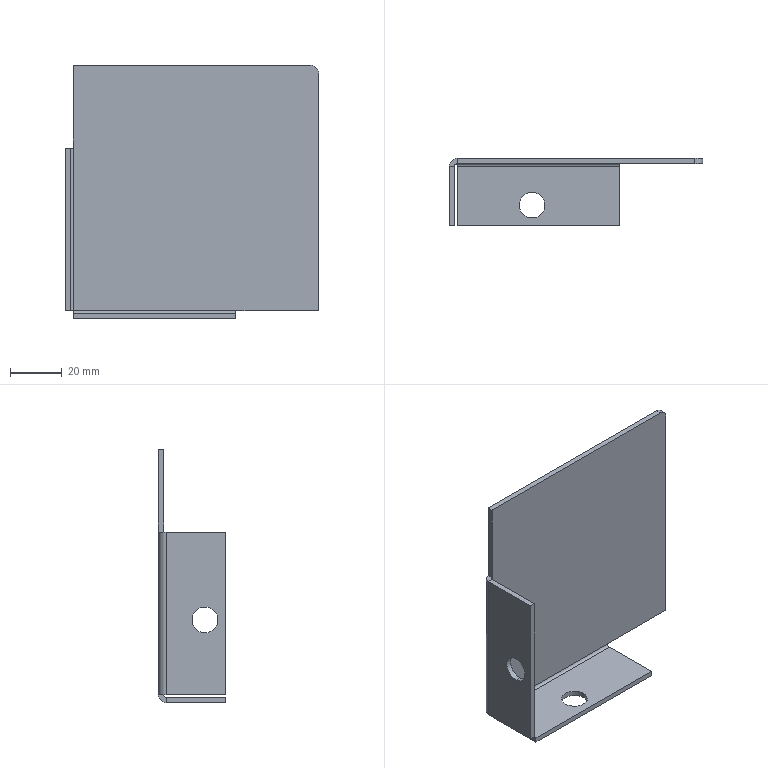Component | SolidWorks | ColumnBlockingPlate-2 | 1 solid | 29 faces | box 98 x 26 x 98 mm | volume 24320 mm3 | plane 20 | cylinder 9 | commonest cylinder face diameters 10 x4 6 x3 2 x2
STEP:
#1=CARTESIAN_POINT('',(85.767,85.53,45.831));
#2=VERTEX_POINT('',#1);
#3=CARTESIAN_POINT('',(85.767,85.53,46.225));
#4=VERTEX_POINT('',#3);
#5=CARTESIAN_POINT('',(85.767,85.53,46.028));
#6=DIRECTION('',(-1.,0.,0.));
#7=DIRECTION('',(0.,-1.,0.));
#8=AXIS2_PLACEMENT_3D('',#5,#6,#7);
#9=CIRCLE('',#8,0.1969);
#10=EDGE_CURVE('',#2,#4,#9,.T.);
#11=ORIENTED_EDGE('',*,*,#10,.F.);
#12=CARTESIAN_POINT('',(85.688,85.53,45.831));
#13=VERTEX_POINT('',#12);
#14=CARTESIAN_POINT('',(85.688,85.53,45.831));
#15=DIRECTION('',(-1.,0.,0.));
#16=VECTOR('',#15,39.37);
#17=LINE('',#14,#16);
#18=EDGE_CURVE('',#2,#13,#17,.T.);
#19=ORIENTED_EDGE('',*,*,#18,.T.);
#20=CARTESIAN_POINT('',(85.688,85.53,46.225));
#21=VERTEX_POINT('',#20);
#22=CARTESIAN_POINT('',(85.688,85.53,46.028));
#23=DIRECTION('',(-1.,0.,0.));
#24=DIRECTION('',(0.,0.,1.));
#25=AXIS2_PLACEMENT_3D('',#22,#23,#24);
#26=CIRCLE('',#25,0.1969);
#27=EDGE_CURVE('',#13,#21,#26,.T.);
#28=ORIENTED_EDGE('',*,*,#27,.T.);
#29=CARTESIAN_POINT('',(85.688,85.53,46.225));
#30=DIRECTION('',(-1.,0.,0.));
#31=VECTOR('',#30,39.37);
#32=LINE('',#29,#31);
#33=EDGE_CURVE('',#4,#21,#32,.T.);
#34=ORIENTED_EDGE('',*,*,#33,.F.);
#35=EDGE_LOOP('',(#11,#19,#28,#34));
#36=FACE_OUTER_BOUND('',#35,.T.);
#37=CARTESIAN_POINT('',(85.688,85.53,46.028));
#38=DIRECTION('',(-1.,0.,0.));
#39=DIRECTION('',(0.,0.,1.));
#40=AXIS2_PLACEMENT_3D('',#37,#38,#39);
#41=CYLINDRICAL_SURFACE('',#40,0.1969);
#42=ADVANCED_FACE('',(#36),#41,.F.);
#43=CARTESIAN_POINT('',(87.145,85.53,44.847));
#44=VERTEX_POINT('',#43);
#45=CARTESIAN_POINT('',(86.751,85.53,44.847));
#46=VERTEX_POINT('',#45);
#47=CARTESIAN_POINT('',(86.948,85.53,44.847));
#48=DIRECTION('',(-0.,0.,-1.));
#49=DIRECTION('',(0.,-1.,0.));
#50=AXIS2_PLACEMENT_3D('',#47,#48,#49);
#51=CIRCLE('',#50,0.1969);
#52=EDGE_CURVE('',#44,#46,#51,.T.);
#53=ORIENTED_EDGE('',*,*,#52,.F.);
#54=CARTESIAN_POINT('',(87.145,85.53,44.768));
#55=VERTEX_POINT('',#54);
#56=CARTESIAN_POINT('',(87.145,85.53,44.768));
#57=DIRECTION('',(-0.,0.,-1.));
#58=VECTOR('',#57,39.37);
#59=LINE('',#56,#58);
#60=EDGE_CURVE('',#44,#55,#59,.T.);
#61=ORIENTED_EDGE('',*,*,#60,.T.);
#62=CARTESIAN_POINT('',(86.751,85.53,44.768));
#63=VERTEX_POINT('',#62);
#64=CARTESIAN_POINT('',(86.948,85.53,44.768));
#65=DIRECTION('',(-0.,0.,-1.));
#66=DIRECTION('',(-1.,0.,0.));
#67=AXIS2_PLACEMENT_3D('',#64,#65,#66);
#68=CIRCLE('',#67,0.1969);
#69=EDGE_CURVE('',#55,#63,#68,.T.);
#70=ORIENTED_EDGE('',*,*,#69,.T.);
#71=CARTESIAN_POINT('',(86.751,85.53,44.768));
#72=DIRECTION('',(-0.,0.,-1.));
#73=VECTOR('',#72,39.37);
#74=LINE('',#71,#73);
#75=EDGE_CURVE('',#46,#63,#74,.T.);
#76=ORIENTED_EDGE('',*,*,#75,.F.);
#77=EDGE_LOOP('',(#53,#61,#70,#76));
#78=FACE_OUTER_BOUND('',#77,.T.);
#79=CARTESIAN_POINT('',(86.948,85.53,44.768));
#80=DIRECTION('',(-0.,0.,-1.));
#81=DIRECTION('',(-1.,0.,0.));
#82=AXIS2_PLACEMENT_3D('',#79,#80,#81);
#83=CYLINDRICAL_SURFACE('',#82,0.1969);
#84=ADVANCED_FACE('',(#78),#83,.F.);
#85=CARTESIAN_POINT('',(85.806,86.239,44.886));
#86=VERTEX_POINT('',#85);
#87=CARTESIAN_POINT('',(85.806,86.239,47.366));
#88=VERTEX_POINT('',#87);
#89=CARTESIAN_POINT('',(85.806,86.239,44.768));
#90=DIRECTION('',(0.,0.,1.));
#91=VECTOR('',#90,39.37);
#92=LINE('',#89,#91);
#93=EDGE_CURVE('',#86,#88,#92,.T.);
#94=ORIENTED_EDGE('',*,*,#93,.F.);
#95=CARTESIAN_POINT('',(85.688,86.12,44.886));
#96=VERTEX_POINT('',#95);
#97=CARTESIAN_POINT('',(85.806,86.12,44.886));
#98=DIRECTION('',(0.,0.,1.));
#99=DIRECTION('',(-1.,0.,0.));
#100=AXIS2_PLACEMENT_3D('',#97,#98,#99);
#101=CIRCLE('',#100,0.1181);
#102=EDGE_CURVE('',#86,#96,#101,.T.);
#103=ORIENTED_EDGE('',*,*,#102,.T.);
#104=CARTESIAN_POINT('',(85.688,86.12,47.366));
#105=VERTEX_POINT('',#104);
#106=CARTESIAN_POINT('',(85.688,86.12,44.768));
#107=DIRECTION('',(-0.,0.,-1.));
#108=VECTOR('',#107,39.37);
#109=LINE('',#106,#108);
#110=EDGE_CURVE('',#105,#96,#109,.T.);
#111=ORIENTED_EDGE('',*,*,#110,.F.);
#112=CARTESIAN_POINT('',(85.806,86.12,47.366));
#113=DIRECTION('',(0.,0.,1.));
#114=DIRECTION('',(1.,0.,0.));
#115=AXIS2_PLACEMENT_3D('',#112,#113,#114);
#116=CIRCLE('',#115,0.1181);
#117=EDGE_CURVE('',#88,#105,#116,.T.);
#118=ORIENTED_EDGE('',*,*,#117,.F.);
#119=EDGE_LOOP('',(#94,#103,#111,#118));
#120=FACE_OUTER_BOUND('',#119,.T.);
#121=CARTESIAN_POINT('',(85.806,86.12,44.768));
#122=DIRECTION('',(-0.,0.,-1.));
#123=DIRECTION('',(-1.,0.,0.));
#124=AXIS2_PLACEMENT_3D('',#121,#122,#123);
#125=CYLINDRICAL_SURFACE('',#124,0.1181);
#126=ADVANCED_FACE('',(#120),#125,.T.);
#127=CARTESIAN_POINT('',(85.806,86.16,44.886));
#128=VERTEX_POINT('',#127);
#129=CARTESIAN_POINT('',(85.767,86.12,44.886));
#130=VERTEX_POINT('',#129);
#131=CARTESIAN_POINT('',(85.806,86.12,44.886));
#132=DIRECTION('',(0.,-0.,1.));
#133=DIRECTION('',(0.,1.,0.));
#134=AXIS2_PLACEMENT_3D('',#131,#132,#133);
#135=CIRCLE('',#134,0.03937);
#136=EDGE_CURVE('',#128,#130,#135,.T.);
#137=ORIENTED_EDGE('',*,*,#136,.F.);
#138=CARTESIAN_POINT('',(85.806,86.16,47.366));
#139=VERTEX_POINT('',#138);
#140=CARTESIAN_POINT('',(85.806,86.16,44.768));
#141=DIRECTION('',(0.,0.,1.));
#142=VECTOR('',#141,39.37);
#143=LINE('',#140,#142);
#144=EDGE_CURVE('',#128,#139,#143,.T.);
#145=ORIENTED_EDGE('',*,*,#144,.T.);
#146=CARTESIAN_POINT('',(85.767,86.12,47.366));
#147=VERTEX_POINT('',#146);
#148=CARTESIAN_POINT('',(85.806,86.12,47.366));
#149=DIRECTION('',(-0.,0.,-1.));
#150=DIRECTION('',(1.,0.,0.));
#151=AXIS2_PLACEMENT_3D('',#148,#149,#150);
#152=CIRCLE('',#151,0.03937);
#153=EDGE_CURVE('',#147,#139,#152,.T.);
#154=ORIENTED_EDGE('',*,*,#153,.F.);
#155=CARTESIAN_POINT('',(85.767,86.12,48.626));
#156=DIRECTION('',(-0.,0.,-1.));
#157=VECTOR('',#156,39.37);
#158=LINE('',#155,#157);
#159=EDGE_CURVE('',#147,#130,#158,.T.);
#160=ORIENTED_EDGE('',*,*,#159,.T.);
#161=EDGE_LOOP('',(#137,#145,#154,#160));
#162=FACE_OUTER_BOUND('',#161,.T.);
#163=CARTESIAN_POINT('',(85.806,86.12,44.768));
#164=DIRECTION('',(-0.,0.,-1.));
#165=DIRECTION('',(-1.,0.,0.));
#166=AXIS2_PLACEMENT_3D('',#163,#164,#165);
#167=CYLINDRICAL_SURFACE('',#166,0.03937);
#168=ADVANCED_FACE('',(#162),#167,.F.);
#169=CARTESIAN_POINT('',(85.688,85.53,46.028));
#170=DIRECTION('',(-1.,0.,0.));
#171=DIRECTION('',(0.,0.,1.));
#172=AXIS2_PLACEMENT_3D('',#169,#170,#171);
#173=CIRCLE('',#172,0.1969);
#174=EDGE_CURVE('',#21,#13,#173,.T.);
#175=ORIENTED_EDGE('',*,*,#174,.F.);
#176=ORIENTED_EDGE('',*,*,#27,.F.);
#177=EDGE_LOOP('',(#175,#176));
#178=FACE_BOUND('',#177,.T.);
#179=ORIENTED_EDGE('',*,*,#110,.T.);
#180=CARTESIAN_POINT('',(85.688,85.215,44.886));
#181=VERTEX_POINT('',#180);
#182=CARTESIAN_POINT('',(85.688,86.16,44.886));
#183=DIRECTION('',(-0.,-1.,0.));
#184=VECTOR('',#183,39.37);
#185=LINE('',#182,#184);
#186=EDGE_CURVE('',#96,#181,#185,.T.);
#187=ORIENTED_EDGE('',*,*,#186,.T.);
#188=CARTESIAN_POINT('',(85.688,85.215,47.366));
#189=VERTEX_POINT('',#188);
#190=CARTESIAN_POINT('',(85.688,85.215,44.768));
#191=DIRECTION('',(-0.,0.,-1.));
#192=VECTOR('',#191,39.37);
#193=LINE('',#190,#192);
#194=EDGE_CURVE('',#189,#181,#193,.T.);
#195=ORIENTED_EDGE('',*,*,#194,.F.);
#196=CARTESIAN_POINT('',(85.688,86.12,47.366));
#197=DIRECTION('',(-0.,-1.,0.));
#198=VECTOR('',#197,39.37);
#199=LINE('',#196,#198);
#200=EDGE_CURVE('',#105,#189,#199,.T.);
#201=ORIENTED_EDGE('',*,*,#200,.F.);
#202=EDGE_LOOP('',(#179,#187,#195,#201));
#203=FACE_OUTER_BOUND('',#202,.T.);
#204=CARTESIAN_POINT('',(85.688,86.16,44.768));
#205=DIRECTION('',(-1.,0.,0.));
#206=DIRECTION('',(-0.,-1.,0.));
#207=AXIS2_PLACEMENT_3D('',#204,#205,#206);
#208=PLANE('',#207);
#209=ADVANCED_FACE('',(#178,#203),#208,.T.);
#210=CARTESIAN_POINT('',(85.767,85.53,46.028));
#211=DIRECTION('',(-1.,0.,0.));
#212=DIRECTION('',(0.,-1.,0.));
#213=AXIS2_PLACEMENT_3D('',#210,#211,#212);
#214=CIRCLE('',#213,0.1969);
#215=EDGE_CURVE('',#4,#2,#214,.T.);
#216=ORIENTED_EDGE('',*,*,#215,.T.);
#217=ORIENTED_EDGE('',*,*,#10,.T.);
#218=EDGE_LOOP('',(#216,#217));
#219=FACE_BOUND('',#218,.T.);
#220=CARTESIAN_POINT('',(85.767,85.215,44.886));
#221=VERTEX_POINT('',#220);
#222=CARTESIAN_POINT('',(85.767,86.12,44.886));
#223=DIRECTION('',(-0.,-1.,-0.));
#224=VECTOR('',#223,39.37);
#225=LINE('',#222,#224);
#226=EDGE_CURVE('',#130,#221,#225,.T.);
#227=ORIENTED_EDGE('',*,*,#226,.F.);
#228=ORIENTED_EDGE('',*,*,#159,.F.);
#229=CARTESIAN_POINT('',(85.767,85.215,47.366));
#230=VERTEX_POINT('',#229);
#231=CARTESIAN_POINT('',(85.767,85.215,47.366));
#232=DIRECTION('',(0.,1.,-0.));
#233=VECTOR('',#232,39.37);
#234=LINE('',#231,#233);
#235=EDGE_CURVE('',#230,#147,#234,.T.);
#236=ORIENTED_EDGE('',*,*,#235,.F.);
#237=CARTESIAN_POINT('',(85.767,85.215,44.768));
#238=DIRECTION('',(-0.,0.,-1.));
#239=VECTOR('',#238,39.37);
#240=LINE('',#237,#239);
#241=EDGE_CURVE('',#230,#221,#240,.T.);
#242=ORIENTED_EDGE('',*,*,#241,.T.);
#243=EDGE_LOOP('',(#227,#228,#236,#242));
#244=FACE_OUTER_BOUND('',#243,.T.);
#245=CARTESIAN_POINT('',(85.767,86.16,44.768));
#246=DIRECTION('',(-1.,0.,0.));
#247=DIRECTION('',(-0.,-1.,0.));
#248=AXIS2_PLACEMENT_3D('',#245,#246,#247);
#249=PLANE('',#248);
#250=ADVANCED_FACE('',(#219,#244),#249,.F.);
#251=ORIENTED_EDGE('',*,*,#194,.T.);
#252=CARTESIAN_POINT('',(85.767,85.215,44.886));
#253=DIRECTION('',(-1.,0.,0.));
#254=VECTOR('',#253,39.37);
#255=LINE('',#252,#254);
#256=EDGE_CURVE('',#221,#181,#255,.T.);
#257=ORIENTED_EDGE('',*,*,#256,.F.);
#258=ORIENTED_EDGE('',*,*,#241,.F.);
#259=CARTESIAN_POINT('',(85.688,85.215,47.366));
#260=DIRECTION('',(1.,-0.,-0.));
#261=VECTOR('',#260,39.37);
#262=LINE('',#259,#261);
#263=EDGE_CURVE('',#189,#230,#262,.T.);
#264=ORIENTED_EDGE('',*,*,#263,.F.);
#265=EDGE_LOOP('',(#251,#257,#258,#264));
#266=FACE_OUTER_BOUND('',#265,.T.);
#267=CARTESIAN_POINT('',(85.688,85.215,44.768));
#268=DIRECTION('',(-0.,-1.,0.));
#269=DIRECTION('',(1.,-0.,-0.));
#270=AXIS2_PLACEMENT_3D('',#267,#268,#269);
#271=PLANE('',#270);
#272=ADVANCED_FACE('',(#266),#271,.T.);
#273=ORIENTED_EDGE('',*,*,#235,.T.);
#274=CARTESIAN_POINT('',(85.767,86.12,47.366));
#275=DIRECTION('',(-1.,0.,0.));
#276=VECTOR('',#275,39.37);
#277=LINE('',#274,#276);
#278=EDGE_CURVE('',#147,#105,#277,.T.);
#279=ORIENTED_EDGE('',*,*,#278,.T.);
#280=ORIENTED_EDGE('',*,*,#200,.T.);
#281=ORIENTED_EDGE('',*,*,#263,.T.);
#282=EDGE_LOOP('',(#273,#279,#280,#281));
#283=FACE_OUTER_BOUND('',#282,.T.);
#284=CARTESIAN_POINT('',(85.806,86.12,47.366));
#285=DIRECTION('',(0.,0.,1.));
#286=DIRECTION('',(1.,0.,-0.));
#287=AXIS2_PLACEMENT_3D('',#284,#285,#286);
#288=PLANE('',#287);
#289=ADVANCED_FACE('',(#283),#288,.T.);
#290=CARTESIAN_POINT('',(88.286,85.215,44.768));
#291=VERTEX_POINT('',#290);
#292=CARTESIAN_POINT('',(88.286,86.12,44.768));
#293=VERTEX_POINT('',#292);
#294=CARTESIAN_POINT('',(88.286,85.215,44.768));
#295=DIRECTION('',(0.,1.,0.));
#296=VECTOR('',#295,39.37);
#297=LINE('',#294,#296);
#298=EDGE_CURVE('',#291,#293,#297,.T.);
#299=ORIENTED_EDGE('',*,*,#298,.T.);
#300=CARTESIAN_POINT('',(88.286,86.12,44.847));
#301=VERTEX_POINT('',#300);
#302=CARTESIAN_POINT('',(88.286,86.12,44.768));
#303=DIRECTION('',(0.,-0.,1.));
#304=VECTOR('',#303,39.37);
#305=LINE('',#302,#304);
#306=EDGE_CURVE('',#293,#301,#305,.T.);
#307=ORIENTED_EDGE('',*,*,#306,.T.);
#308=CARTESIAN_POINT('',(88.286,85.215,44.847));
#309=VERTEX_POINT('',#308);
#310=CARTESIAN_POINT('',(88.286,86.12,44.847));
#311=DIRECTION('',(-0.,-1.,-0.));
#312=VECTOR('',#311,39.37);
#313=LINE('',#310,#312);
#314=EDGE_CURVE('',#301,#309,#313,.T.);
#315=ORIENTED_EDGE('',*,*,#314,.T.);
#316=CARTESIAN_POINT('',(88.286,85.215,44.847));
#317=DIRECTION('',(-0.,0.,-1.));
#318=VECTOR('',#317,39.37);
#319=LINE('',#316,#318);
#320=EDGE_CURVE('',#309,#291,#319,.T.);
#321=ORIENTED_EDGE('',*,*,#320,.T.);
#322=EDGE_LOOP('',(#299,#307,#315,#321));
#323=FACE_OUTER_BOUND('',#322,.T.);
#324=CARTESIAN_POINT('',(88.286,86.12,44.886));
#325=DIRECTION('',(1.,0.,-0.));
#326=DIRECTION('',(-0.,0.,-1.));
#327=AXIS2_PLACEMENT_3D('',#324,#325,#326);
#328=PLANE('',#327);
#329=ADVANCED_FACE('',(#323),#328,.T.);
#330=CARTESIAN_POINT('',(88.286,86.239,44.886));
#331=VERTEX_POINT('',#330);
#332=CARTESIAN_POINT('',(89.546,86.239,44.886));
#333=DIRECTION('',(-1.,0.,0.));
#334=VECTOR('',#333,39.37);
#335=LINE('',#332,#334);
#336=EDGE_CURVE('',#331,#86,#335,.T.);
#337=ORIENTED_EDGE('',*,*,#336,.F.);
#338=CARTESIAN_POINT('',(88.286,86.12,44.886));
#339=DIRECTION('',(1.,0.,-0.));
#340=DIRECTION('',(0.,0.,-1.));
#341=AXIS2_PLACEMENT_3D('',#338,#339,#340);
#342=CIRCLE('',#341,0.1181);
#343=EDGE_CURVE('',#293,#331,#342,.T.);
#344=ORIENTED_EDGE('',*,*,#343,.F.);
#345=CARTESIAN_POINT('',(85.806,86.12,44.768));
#346=VERTEX_POINT('',#345);
#347=CARTESIAN_POINT('',(89.546,86.12,44.768));
#348=DIRECTION('',(1.,0.,-0.));
#349=VECTOR('',#348,39.37);
#350=LINE('',#347,#349);
#351=EDGE_CURVE('',#346,#293,#350,.T.);
#352=ORIENTED_EDGE('',*,*,#351,.F.);
#353=CARTESIAN_POINT('',(85.806,86.12,44.886));
#354=DIRECTION('',(-1.,0.,0.));
#355=DIRECTION('',(0.,0.,-1.));
#356=AXIS2_PLACEMENT_3D('',#353,#354,#355);
#357=CIRCLE('',#356,0.1181);
#358=EDGE_CURVE('',#86,#346,#357,.T.);
#359=ORIENTED_EDGE('',*,*,#358,.F.);
#360=EDGE_LOOP('',(#337,#344,#352,#359));
#361=FACE_OUTER_BOUND('',#360,.T.);
#362=CARTESIAN_POINT('',(89.546,86.12,44.886));
#363=DIRECTION('',(1.,0.,-0.));
#364=DIRECTION('',(0.,0.,-1.));
#365=AXIS2_PLACEMENT_3D('',#362,#363,#364);
#366=CYLINDRICAL_SURFACE('',#365,0.1181);
#367=ADVANCED_FACE('',(#361),#366,.T.);
#368=CARTESIAN_POINT('',(88.286,86.16,44.886));
#369=VERTEX_POINT('',#368);
#370=CARTESIAN_POINT('',(88.286,86.12,44.886));
#371=DIRECTION('',(-1.,0.,0.));
#372=DIRECTION('',(0.,0.,-1.));
#373=AXIS2_PLACEMENT_3D('',#370,#371,#372);
#374=CIRCLE('',#373,0.03937);
#375=EDGE_CURVE('',#369,#301,#374,.T.);
#376=ORIENTED_EDGE('',*,*,#375,.F.);
#377=CARTESIAN_POINT('',(89.546,86.16,44.886));
#378=DIRECTION('',(-1.,0.,0.));
#379=VECTOR('',#378,39.37);
#380=LINE('',#377,#379);
#381=EDGE_CURVE('',#369,#128,#380,.T.);
#382=ORIENTED_EDGE('',*,*,#381,.T.);
#383=CARTESIAN_POINT('',(85.806,86.12,44.847));
#384=VERTEX_POINT('',#383);
#385=CARTESIAN_POINT('',(85.806,86.12,44.886));
#386=DIRECTION('',(-1.,0.,0.));
#387=DIRECTION('',(0.,0.,-1.));
#388=AXIS2_PLACEMENT_3D('',#385,#386,#387);
#389=CIRCLE('',#388,0.03937);
#390=EDGE_CURVE('',#128,#384,#389,.T.);
#391=ORIENTED_EDGE('',*,*,#390,.T.);
#392=CARTESIAN_POINT('',(85.806,86.12,44.847));
#393=DIRECTION('',(1.,0.,-0.));
#394=VECTOR('',#393,39.37);
#395=LINE('',#392,#394);
#396=EDGE_CURVE('',#384,#301,#395,.T.);
#397=ORIENTED_EDGE('',*,*,#396,.T.);
#398=EDGE_LOOP('',(#376,#382,#391,#397));
#399=FACE_OUTER_BOUND('',#398,.T.);
#400=CARTESIAN_POINT('',(89.546,86.12,44.886));
#401=DIRECTION('',(1.,0.,-0.));
#402=DIRECTION('',(0.,0.,-1.));
#403=AXIS2_PLACEMENT_3D('',#400,#401,#402);
#404=CYLINDRICAL_SURFACE('',#403,0.03937);
#405=ADVANCED_FACE('',(#399),#404,.F.);
#406=CARTESIAN_POINT('',(86.948,85.53,44.768));
#407=DIRECTION('',(-0.,0.,-1.));
#408=DIRECTION('',(-1.,0.,0.));
#409=AXIS2_PLACEMENT_3D('',#406,#407,#408);
#410=CIRCLE('',#409,0.1969);
#411=EDGE_CURVE('',#63,#55,#410,.T.);
#412=ORIENTED_EDGE('',*,*,#411,.F.);
#413=ORIENTED_EDGE('',*,*,#69,.F.);
#414=EDGE_LOOP('',(#412,#413));
#415=FACE_BOUND('',#414,.T.);
#416=ORIENTED_EDGE('',*,*,#351,.T.);
#417=ORIENTED_EDGE('',*,*,#298,.F.);
#418=CARTESIAN_POINT('',(85.806,85.215,44.768));
#419=VERTEX_POINT('',#418);
#420=CARTESIAN_POINT('',(89.546,85.215,44.768));
#421=DIRECTION('',(1.,0.,-0.));
#422=VECTOR('',#421,39.37);
#423=LINE('',#420,#422);
#424=EDGE_CURVE('',#419,#291,#423,.T.);
#425=ORIENTED_EDGE('',*,*,#424,.F.);
#426=CARTESIAN_POINT('',(85.806,85.215,44.768));
#427=DIRECTION('',(-0.,-1.,-0.));
#428=VECTOR('',#427,39.37);
#429=LINE('',#426,#428);
#430=EDGE_CURVE('',#346,#419,#429,.T.);
#431=ORIENTED_EDGE('',*,*,#430,.F.);
#432=EDGE_LOOP('',(#416,#417,#425,#431));
#433=FACE_OUTER_BOUND('',#432,.T.);
#434=CARTESIAN_POINT('',(89.546,86.16,44.768));
#435=DIRECTION('',(-0.,0.,-1.));
#436=DIRECTION('',(-0.,-1.,-0.));
#437=AXIS2_PLACEMENT_3D('',#434,#435,#436);
#438=PLANE('',#437);
#439=ADVANCED_FACE('',(#415,#433),#438,.T.);
#440=CARTESIAN_POINT('',(86.948,85.53,44.847));
#441=DIRECTION('',(-0.,0.,-1.));
#442=DIRECTION('',(0.,-1.,0.));
#443=AXIS2_PLACEMENT_3D('',#440,#441,#442);
#444=CIRCLE('',#443,0.1969);
#445=EDGE_CURVE('',#46,#44,#444,.T.);
#446=ORIENTED_EDGE('',*,*,#445,.T.);
#447=ORIENTED_EDGE('',*,*,#52,.T.);
#448=EDGE_LOOP('',(#446,#447));
#449=FACE_BOUND('',#448,.T.);
#450=ORIENTED_EDGE('',*,*,#314,.F.);
#451=ORIENTED_EDGE('',*,*,#396,.F.);
#452=CARTESIAN_POINT('',(85.806,85.215,44.847));
#453=VERTEX_POINT('',#452);
#454=CARTESIAN_POINT('',(85.806,86.16,44.847));
#455=DIRECTION('',(-0.,-1.,-0.));
#456=VECTOR('',#455,39.37);
#457=LINE('',#454,#456);
#458=EDGE_CURVE('',#384,#453,#457,.T.);
#459=ORIENTED_EDGE('',*,*,#458,.T.);
#460=CARTESIAN_POINT('',(89.546,85.215,44.847));
#461=DIRECTION('',(1.,0.,-0.));
#462=VECTOR('',#461,39.37);
#463=LINE('',#460,#462);
#464=EDGE_CURVE('',#453,#309,#463,.T.);
#465=ORIENTED_EDGE('',*,*,#464,.T.);
#466=EDGE_LOOP('',(#450,#451,#459,#465));
#467=FACE_OUTER_BOUND('',#466,.T.);
#468=CARTESIAN_POINT('',(89.546,86.16,44.847));
#469=DIRECTION('',(-0.,0.,-1.));
#470=DIRECTION('',(-0.,-1.,-0.));
#471=AXIS2_PLACEMENT_3D('',#468,#469,#470);
#472=PLANE('',#471);
#473=ADVANCED_FACE('',(#449,#467),#472,.F.);
#474=ORIENTED_EDGE('',*,*,#424,.T.);
#475=ORIENTED_EDGE('',*,*,#320,.F.);
#476=ORIENTED_EDGE('',*,*,#464,.F.);
#477=CARTESIAN_POINT('',(85.806,85.215,44.768));
#478=DIRECTION('',(0.,-0.,1.));
#479=VECTOR('',#478,39.37);
#480=LINE('',#477,#479);
#481=EDGE_CURVE('',#419,#453,#480,.T.);
#482=ORIENTED_EDGE('',*,*,#481,.F.);
#483=EDGE_LOOP('',(#474,#475,#476,#482));
#484=FACE_OUTER_BOUND('',#483,.T.);
#485=CARTESIAN_POINT('',(89.546,85.215,44.768));
#486=DIRECTION('',(-0.,-1.,-0.));
#487=DIRECTION('',(0.,-0.,1.));
#488=AXIS2_PLACEMENT_3D('',#485,#486,#487);
#489=PLANE('',#488);
#490=ADVANCED_FACE('',(#484),#489,.T.);
#491=CARTESIAN_POINT('',(89.546,86.16,48.508));
#492=VERTEX_POINT('',#491);
#493=CARTESIAN_POINT('',(89.546,86.16,44.886));
#494=VERTEX_POINT('',#493);
#495=CARTESIAN_POINT('',(89.546,86.16,44.768));
#496=DIRECTION('',(-0.,0.,-1.));
#497=VECTOR('',#496,39.37);
#498=LINE('',#495,#497);
#499=EDGE_CURVE('',#492,#494,#498,.T.);
#500=ORIENTED_EDGE('',*,*,#499,.F.);
#501=CARTESIAN_POINT('',(89.428,86.16,48.626));
#502=VERTEX_POINT('',#501);
#503=CARTESIAN_POINT('',(89.428,86.16,48.508));
#504=DIRECTION('',(0.,-1.,0.));
#505=DIRECTION('',(1.,0.,0.));
#506=AXIS2_PLACEMENT_3D('',#503,#504,#505);
#507=CIRCLE('',#506,0.1181);
#508=EDGE_CURVE('',#492,#502,#507,.T.);
#509=ORIENTED_EDGE('',*,*,#508,.T.);
#510=CARTESIAN_POINT('',(85.806,86.16,48.626));
#511=VERTEX_POINT('',#510);
#512=CARTESIAN_POINT('',(85.688,86.16,48.626));
#513=DIRECTION('',(1.,0.,-0.));
#514=VECTOR('',#513,39.37);
#515=LINE('',#512,#514);
#516=EDGE_CURVE('',#511,#502,#515,.T.);
#517=ORIENTED_EDGE('',*,*,#516,.F.);
#518=CARTESIAN_POINT('',(85.806,86.16,47.366));
#519=DIRECTION('',(0.,0.,1.));
#520=VECTOR('',#519,39.37);
#521=LINE('',#518,#520);
#522=EDGE_CURVE('',#139,#511,#521,.T.);
#523=ORIENTED_EDGE('',*,*,#522,.F.);
#524=ORIENTED_EDGE('',*,*,#144,.F.);
#525=ORIENTED_EDGE('',*,*,#381,.F.);
#526=CARTESIAN_POINT('',(89.546,86.16,44.886));
#527=DIRECTION('',(-1.,0.,0.));
#528=VECTOR('',#527,39.37);
#529=LINE('',#526,#528);
#530=EDGE_CURVE('',#494,#369,#529,.T.);
#531=ORIENTED_EDGE('',*,*,#530,.F.);
#532=EDGE_LOOP('',(#500,#509,#517,#523,#524,#525,#531));
#533=FACE_OUTER_BOUND('',#532,.T.);
#534=CARTESIAN_POINT('',(89.546,86.16,44.768));
#535=DIRECTION('',(0.,-1.,0.));
#536=DIRECTION('',(1.,0.,-0.));
#537=AXIS2_PLACEMENT_3D('',#534,#535,#536);
#538=PLANE('',#537);
#539=ADVANCED_FACE('',(#533),#538,.T.);
#540=CARTESIAN_POINT('',(85.806,86.239,48.626));
#541=VERTEX_POINT('',#540);
#542=CARTESIAN_POINT('',(89.428,86.239,48.626));
#543=VERTEX_POINT('',#542);
#544=CARTESIAN_POINT('',(85.688,86.239,48.626));
#545=DIRECTION('',(1.,0.,-0.));
#546=VECTOR('',#545,39.37);
#547=LINE('',#544,#546);
#548=EDGE_CURVE('',#541,#543,#547,.T.);
#549=ORIENTED_EDGE('',*,*,#548,.T.);
#550=CARTESIAN_POINT('',(89.546,86.239,48.508));
#551=VERTEX_POINT('',#550);
#552=CARTESIAN_POINT('',(89.428,86.239,48.508));
#553=DIRECTION('',(0.,1.,0.));
#554=DIRECTION('',(1.,0.,0.));
#555=AXIS2_PLACEMENT_3D('',#552,#553,#554);
#556=CIRCLE('',#555,0.1181);
#557=EDGE_CURVE('',#543,#551,#556,.T.);
#558=ORIENTED_EDGE('',*,*,#557,.T.);
#559=CARTESIAN_POINT('',(89.546,86.239,44.886));
#560=VERTEX_POINT('',#559);
#561=CARTESIAN_POINT('',(89.546,86.239,44.768));
#562=DIRECTION('',(-0.,0.,-1.));
#563=VECTOR('',#562,39.37);
#564=LINE('',#561,#563);
#565=EDGE_CURVE('',#551,#560,#564,.T.);
#566=ORIENTED_EDGE('',*,*,#565,.T.);
#567=CARTESIAN_POINT('',(89.546,86.239,44.886));
#568=DIRECTION('',(-1.,0.,0.));
#569=VECTOR('',#568,39.37);
#570=LINE('',#567,#569);
#571=EDGE_CURVE('',#560,#331,#570,.T.);
#572=ORIENTED_EDGE('',*,*,#571,.T.);
#573=ORIENTED_EDGE('',*,*,#336,.T.);
#574=ORIENTED_EDGE('',*,*,#93,.T.);
#575=CARTESIAN_POINT('',(85.806,86.239,47.366));
#576=DIRECTION('',(0.,0.,1.));
#577=VECTOR('',#576,39.37);
#578=LINE('',#575,#577);
#579=EDGE_CURVE('',#88,#541,#578,.T.);
#580=ORIENTED_EDGE('',*,*,#579,.T.);
#581=EDGE_LOOP('',(#549,#558,#566,#572,#573,#574,#580));
#582=FACE_OUTER_BOUND('',#581,.T.);
#583=CARTESIAN_POINT('',(89.546,86.239,44.768));
#584=DIRECTION('',(0.,-1.,0.));
#585=DIRECTION('',(1.,0.,-0.));
#586=AXIS2_PLACEMENT_3D('',#583,#584,#585);
#587=PLANE('',#586);
#588=ADVANCED_FACE('',(#582),#587,.F.);
#589=ORIENTED_EDGE('',*,*,#565,.F.);
#590=CARTESIAN_POINT('',(89.546,86.16,48.508));
#591=DIRECTION('',(0.,-1.,0.));
#592=VECTOR('',#591,39.37);
#593=LINE('',#590,#592);
#594=EDGE_CURVE('',#551,#492,#593,.T.);
#595=ORIENTED_EDGE('',*,*,#594,.T.);
#596=ORIENTED_EDGE('',*,*,#499,.T.);
#597=CARTESIAN_POINT('',(89.546,86.16,44.886));
#598=DIRECTION('',(0.,1.,0.));
#599=VECTOR('',#598,39.37);
#600=LINE('',#597,#599);
#601=EDGE_CURVE('',#494,#560,#600,.T.);
#602=ORIENTED_EDGE('',*,*,#601,.T.);
#603=EDGE_LOOP('',(#589,#595,#596,#602));
#604=FACE_OUTER_BOUND('',#603,.T.);
#605=CARTESIAN_POINT('',(89.546,86.16,44.768));
#606=DIRECTION('',(1.,0.,-0.));
#607=DIRECTION('',(-0.,0.,-1.));
#608=AXIS2_PLACEMENT_3D('',#605,#606,#607);
#609=PLANE('',#608);
#610=ADVANCED_FACE('',(#604),#609,.T.);
#611=ORIENTED_EDGE('',*,*,#516,.T.);
#612=CARTESIAN_POINT('',(89.428,86.16,48.626));
#613=DIRECTION('',(0.,1.,0.));
#614=VECTOR('',#613,39.37);
#615=LINE('',#612,#614);
#616=EDGE_CURVE('',#502,#543,#615,.T.);
#617=ORIENTED_EDGE('',*,*,#616,.T.);
#618=ORIENTED_EDGE('',*,*,#548,.F.);
#619=CARTESIAN_POINT('',(85.806,86.16,48.626));
#620=DIRECTION('',(0.,1.,0.));
#621=VECTOR('',#620,39.37);
#622=LINE('',#619,#621);
#623=EDGE_CURVE('',#511,#541,#622,.T.);
#624=ORIENTED_EDGE('',*,*,#623,.F.);
#625=EDGE_LOOP('',(#611,#617,#618,#624));
#626=FACE_OUTER_BOUND('',#625,.T.);
#627=CARTESIAN_POINT('',(85.688,86.16,48.626));
#628=DIRECTION('',(0.,0.,1.));
#629=DIRECTION('',(1.,0.,-0.));
#630=AXIS2_PLACEMENT_3D('',#627,#628,#629);
#631=PLANE('',#630);
#632=ADVANCED_FACE('',(#626),#631,.T.);
#633=ORIENTED_EDGE('',*,*,#390,.F.);
#634=CARTESIAN_POINT('',(85.806,86.16,44.886));
#635=DIRECTION('',(0.,1.,-0.));
#636=VECTOR('',#635,39.37);
#637=LINE('',#634,#636);
#638=EDGE_CURVE('',#128,#86,#637,.T.);
#639=ORIENTED_EDGE('',*,*,#638,.T.);
#640=ORIENTED_EDGE('',*,*,#358,.T.);
#641=CARTESIAN_POINT('',(85.806,86.12,44.768));
#642=DIRECTION('',(-0.,0.,-1.));
#643=VECTOR('',#642,39.37);
#644=LINE('',#641,#643);
#645=EDGE_CURVE('',#384,#346,#644,.T.);
#646=ORIENTED_EDGE('',*,*,#645,.F.);
#647=EDGE_LOOP('',(#633,#639,#640,#646));
#648=FACE_OUTER_BOUND('',#647,.T.);
#649=CARTESIAN_POINT('',(85.806,86.12,44.886));
#650=DIRECTION('',(-1.,0.,0.));
#651=DIRECTION('',(0.,0.,1.));
#652=AXIS2_PLACEMENT_3D('',#649,#650,#651);
#653=PLANE('',#652);
#654=ADVANCED_FACE('',(#648),#653,.T.);
#655=ORIENTED_EDGE('',*,*,#458,.F.);
#656=ORIENTED_EDGE('',*,*,#645,.T.);
#657=ORIENTED_EDGE('',*,*,#430,.T.);
#658=ORIENTED_EDGE('',*,*,#481,.T.);
#659=EDGE_LOOP('',(#655,#656,#657,#658));
#660=FACE_OUTER_BOUND('',#659,.T.);
#661=CARTESIAN_POINT('',(85.806,85.215,44.768));
#662=DIRECTION('',(-1.,0.,0.));
#663=DIRECTION('',(-0.,-1.,0.));
#664=AXIS2_PLACEMENT_3D('',#661,#662,#663);
#665=PLANE('',#664);
#666=ADVANCED_FACE('',(#660),#665,.T.);
#667=ORIENTED_EDGE('',*,*,#60,.F.);
#668=ORIENTED_EDGE('',*,*,#445,.F.);
#669=ORIENTED_EDGE('',*,*,#75,.T.);
#670=ORIENTED_EDGE('',*,*,#411,.T.);
#671=EDGE_LOOP('',(#667,#668,#669,#670));
#672=FACE_OUTER_BOUND('',#671,.T.);
#673=CARTESIAN_POINT('',(86.948,85.53,44.768));
#674=DIRECTION('',(-0.,0.,-1.));
#675=DIRECTION('',(-1.,0.,0.));
#676=AXIS2_PLACEMENT_3D('',#673,#674,#675);
#677=CYLINDRICAL_SURFACE('',#676,0.1969);
#678=ADVANCED_FACE('',(#672),#677,.F.);
#679=ORIENTED_EDGE('',*,*,#18,.F.);
#680=ORIENTED_EDGE('',*,*,#215,.F.);
#681=ORIENTED_EDGE('',*,*,#33,.T.);
#682=ORIENTED_EDGE('',*,*,#174,.T.);
#683=EDGE_LOOP('',(#679,#680,#681,#682));
#684=FACE_OUTER_BOUND('',#683,.T.);
#685=CARTESIAN_POINT('',(85.688,85.53,46.028));
#686=DIRECTION('',(-1.,0.,0.));
#687=DIRECTION('',(0.,0.,1.));
#688=AXIS2_PLACEMENT_3D('',#685,#686,#687);
#689=CYLINDRICAL_SURFACE('',#688,0.1969);
#690=ADVANCED_FACE('',(#684),#689,.F.);
#691=ORIENTED_EDGE('',*,*,#601,.F.);
#692=ORIENTED_EDGE('',*,*,#530,.T.);
#693=CARTESIAN_POINT('',(88.286,86.239,44.886));
#694=DIRECTION('',(-0.,-1.,-0.));
#695=VECTOR('',#694,39.37);
#696=LINE('',#693,#695);
#697=EDGE_CURVE('',#331,#369,#696,.T.);
#698=ORIENTED_EDGE('',*,*,#697,.F.);
#699=ORIENTED_EDGE('',*,*,#571,.F.);
#700=EDGE_LOOP('',(#691,#692,#698,#699));
#701=FACE_OUTER_BOUND('',#700,.T.);
#702=CARTESIAN_POINT('',(88.286,86.239,44.886));
#703=DIRECTION('',(0.,-0.,1.));
#704=DIRECTION('',(0.,1.,0.));
#705=AXIS2_PLACEMENT_3D('',#702,#703,#704);
#706=PLANE('',#705);
#707=ADVANCED_FACE('',(#701),#706,.F.);
#708=ORIENTED_EDGE('',*,*,#306,.F.);
#709=ORIENTED_EDGE('',*,*,#343,.T.);
#710=ORIENTED_EDGE('',*,*,#697,.T.);
#711=ORIENTED_EDGE('',*,*,#375,.T.);
#712=EDGE_LOOP('',(#708,#709,#710,#711));
#713=FACE_OUTER_BOUND('',#712,.T.);
#714=CARTESIAN_POINT('',(88.286,86.12,44.886));
#715=DIRECTION('',(1.,0.,-0.));
#716=DIRECTION('',(-0.,0.,-1.));
#717=AXIS2_PLACEMENT_3D('',#714,#715,#716);
#718=PLANE('',#717);
#719=ADVANCED_FACE('',(#713),#718,.T.);
#720=ORIENTED_EDGE('',*,*,#623,.T.);
#721=ORIENTED_EDGE('',*,*,#579,.F.);
#722=CARTESIAN_POINT('',(85.806,86.16,47.366));
#723=DIRECTION('',(0.,1.,0.));
#724=VECTOR('',#723,39.37);
#725=LINE('',#722,#724);
#726=EDGE_CURVE('',#139,#88,#725,.T.);
#727=ORIENTED_EDGE('',*,*,#726,.F.);
#728=ORIENTED_EDGE('',*,*,#522,.T.);
#729=EDGE_LOOP('',(#720,#721,#727,#728));
#730=FACE_OUTER_BOUND('',#729,.T.);
#731=CARTESIAN_POINT('',(85.806,86.16,47.366));
#732=DIRECTION('',(1.,0.,-0.));
#733=DIRECTION('',(-0.,0.,-1.));
#734=AXIS2_PLACEMENT_3D('',#731,#732,#733);
#735=PLANE('',#734);
#736=ADVANCED_FACE('',(#730),#735,.F.);
#737=ORIENTED_EDGE('',*,*,#278,.F.);
#738=ORIENTED_EDGE('',*,*,#153,.T.);
#739=ORIENTED_EDGE('',*,*,#726,.T.);
#740=ORIENTED_EDGE('',*,*,#117,.T.);
#741=EDGE_LOOP('',(#737,#738,#739,#740));
#742=FACE_OUTER_BOUND('',#741,.T.);
#743=CARTESIAN_POINT('',(85.806,86.12,47.366));
#744=DIRECTION('',(0.,0.,1.));
#745=DIRECTION('',(1.,0.,-0.));
#746=AXIS2_PLACEMENT_3D('',#743,#744,#745);
#747=PLANE('',#746);
#748=ADVANCED_FACE('',(#742),#747,.T.);
#749=CARTESIAN_POINT('',(85.767,86.12,44.886));
#750=DIRECTION('',(-1.,0.,0.));
#751=VECTOR('',#750,39.37);
#752=LINE('',#749,#751);
#753=EDGE_CURVE('',#130,#96,#752,.T.);
#754=ORIENTED_EDGE('',*,*,#753,.F.);
#755=ORIENTED_EDGE('',*,*,#226,.T.);
#756=ORIENTED_EDGE('',*,*,#256,.T.);
#757=ORIENTED_EDGE('',*,*,#186,.F.);
#758=EDGE_LOOP('',(#754,#755,#756,#757));
#759=FACE_OUTER_BOUND('',#758,.T.);
#760=CARTESIAN_POINT('',(85.767,86.12,44.886));
#761=DIRECTION('',(-0.,0.,-1.));
#762=DIRECTION('',(-0.,-1.,-0.));
#763=AXIS2_PLACEMENT_3D('',#760,#761,#762);
#764=PLANE('',#763);
#765=ADVANCED_FACE('',(#759),#764,.T.);
#766=ORIENTED_EDGE('',*,*,#638,.F.);
#767=ORIENTED_EDGE('',*,*,#136,.T.);
#768=ORIENTED_EDGE('',*,*,#753,.T.);
#769=ORIENTED_EDGE('',*,*,#102,.F.);
#770=EDGE_LOOP('',(#766,#767,#768,#769));
#771=FACE_OUTER_BOUND('',#770,.T.);
#772=CARTESIAN_POINT('',(85.806,86.12,44.886));
#773=DIRECTION('',(-0.,0.,-1.));
#774=DIRECTION('',(-0.,-1.,-0.));
#775=AXIS2_PLACEMENT_3D('',#772,#773,#774);
#776=PLANE('',#775);
#777=ADVANCED_FACE('',(#771),#776,.T.);
#778=ORIENTED_EDGE('',*,*,#508,.F.);
#779=ORIENTED_EDGE('',*,*,#594,.F.);
#780=ORIENTED_EDGE('',*,*,#557,.F.);
#781=ORIENTED_EDGE('',*,*,#616,.F.);
#782=EDGE_LOOP('',(#778,#779,#780,#781));
#783=FACE_OUTER_BOUND('',#782,.T.);
#784=CARTESIAN_POINT('',(89.428,86.16,48.508));
#785=DIRECTION('',(0.,1.,0.));
#786=DIRECTION('',(-1.,0.,0.));
#787=AXIS2_PLACEMENT_3D('',#784,#785,#786);
#788=CYLINDRICAL_SURFACE('',#787,0.1181);
#789=ADVANCED_FACE('',(#783),#788,.T.);
#790=CLOSED_SHELL('',(#42,#84,#126,#168,#209,#250,#272,#289,#329,#367,#405,#439,#473,#490,#539,#588,#610,#632,#654,#666,#678,#690,#707,#719,#736,#748,#765,#777,#789));
#791=MANIFOLD_SOLID_BREP('',#790);
#792=CARTESIAN_POINT('',(0.,0.,0.));
#793=DIRECTION('',(0.,0.,1.));
#794=DIRECTION('',(1.,0.,0.));
#795=AXIS2_PLACEMENT_3D('',#792,#793,#794);
#796=(LENGTH_UNIT()NAMED_UNIT(*)SI_UNIT($,.METRE.));
#797=LENGTH_MEASURE_WITH_UNIT(LENGTH_MEASURE(0.0254),#796);
#798=DIMENSIONAL_EXPONENTS(1.,0.,0.,0.,0.,0.,0.);
#799=(CONVERSION_BASED_UNIT('',#797)LENGTH_UNIT()NAMED_UNIT(#798));
#800=UNCERTAINTY_MEASURE_WITH_UNIT(LENGTH_MEASURE(0.00001),#799,'','');
#801=(NAMED_UNIT(*)PLANE_ANGLE_UNIT()SI_UNIT($,.RADIAN.));
#802=(NAMED_UNIT(*)SI_UNIT($,.STERADIAN.)SOLID_ANGLE_UNIT());
#803=(GEOMETRIC_REPRESENTATION_CONTEXT(3)GLOBAL_UNCERTAINTY_ASSIGNED_CONTEXT((#800))GLOBAL_UNIT_ASSIGNED_CONTEXT((#799,#801,#802))REPRESENTATION_CONTEXT('',''));
#804=ADVANCED_BREP_SHAPE_REPRESENTATION('',(#791,#795),#803);
#805=COLOUR_RGB('',0.7922,0.8196,0.9333);
#806=FILL_AREA_STYLE_COLOUR('',#805);
#807=FILL_AREA_STYLE('',(#806));
#808=SURFACE_STYLE_FILL_AREA(#807);
#809=SURFACE_SIDE_STYLE('',(#808));
#810=SURFACE_STYLE_USAGE(.BOTH.,#809);
#811=PRESENTATION_STYLE_ASSIGNMENT((#810));
#812=STYLED_ITEM('',(#811),#791);
#813=PRESENTATION_LAYER_ASSIGNMENT('','',(#812));
#814=(LENGTH_UNIT()NAMED_UNIT(*)SI_UNIT($,.METRE.));
#815=LENGTH_MEASURE_WITH_UNIT(LENGTH_MEASURE(0.0254),#814);
#816=DIMENSIONAL_EXPONENTS(1.,0.,0.,0.,0.,0.,0.);
#817=(CONVERSION_BASED_UNIT('',#815)LENGTH_UNIT()NAMED_UNIT(#816));
#818=UNCERTAINTY_MEASURE_WITH_UNIT(LENGTH_MEASURE(0.00001),#817,'','');
#819=(NAMED_UNIT(*)PLANE_ANGLE_UNIT()SI_UNIT($,.RADIAN.));
#820=(NAMED_UNIT(*)SI_UNIT($,.STERADIAN.)SOLID_ANGLE_UNIT());
#821=(GEOMETRIC_REPRESENTATION_CONTEXT(3)GLOBAL_UNCERTAINTY_ASSIGNED_CONTEXT((#818))GLOBAL_UNIT_ASSIGNED_CONTEXT((#817,#819,#820))REPRESENTATION_CONTEXT('',''));
#822=MECHANICAL_DESIGN_GEOMETRIC_PRESENTATION_REPRESENTATION('',(#812),#821);